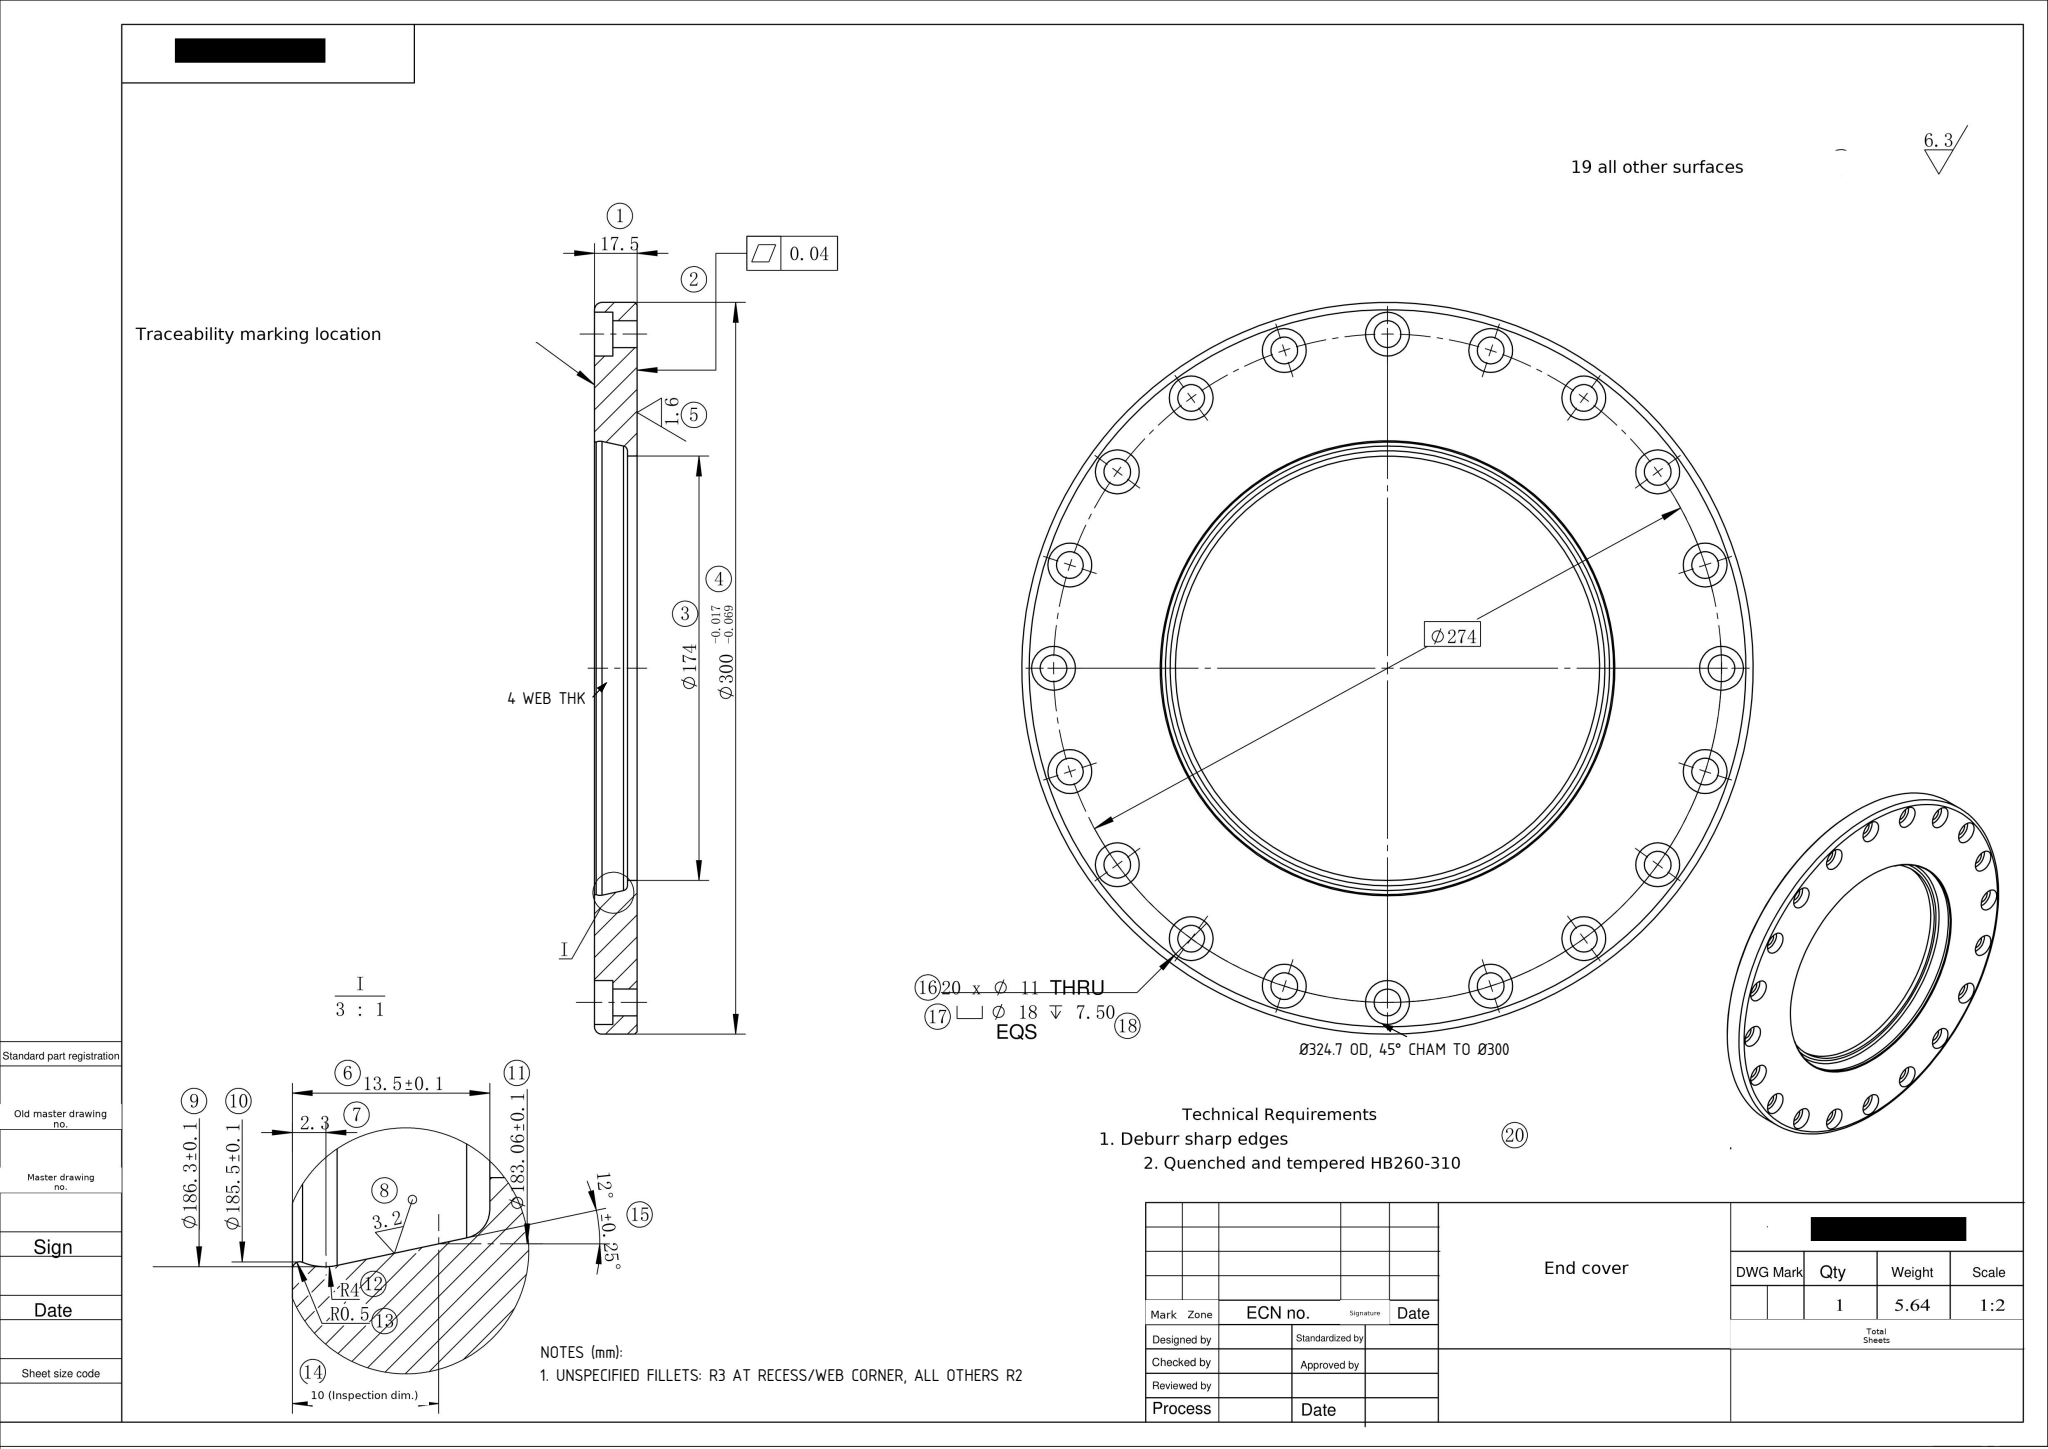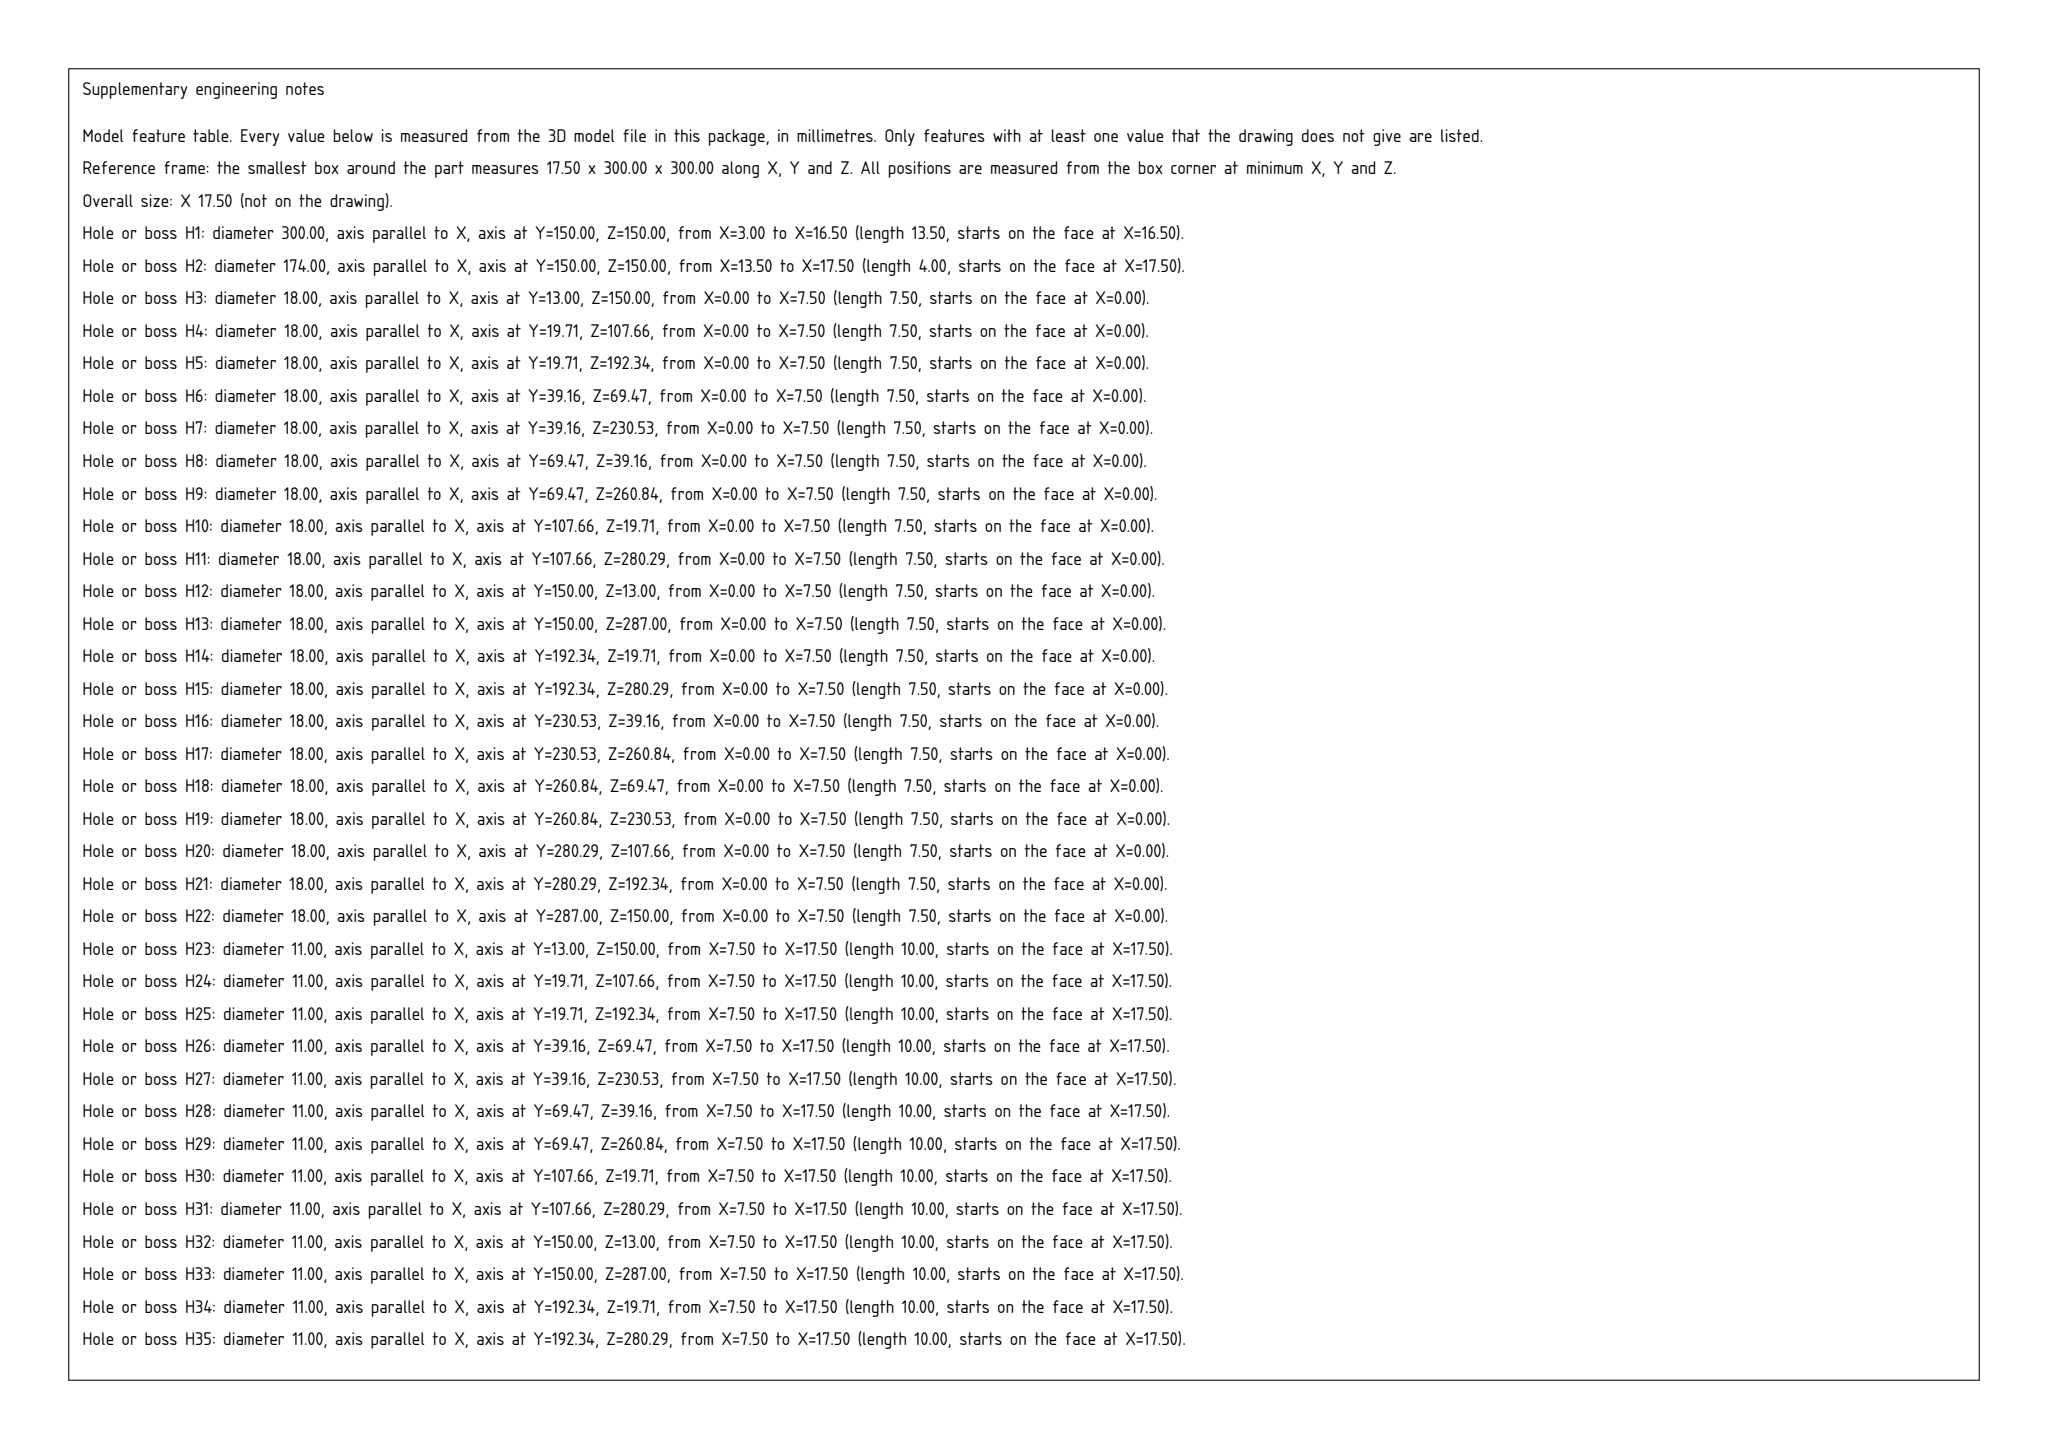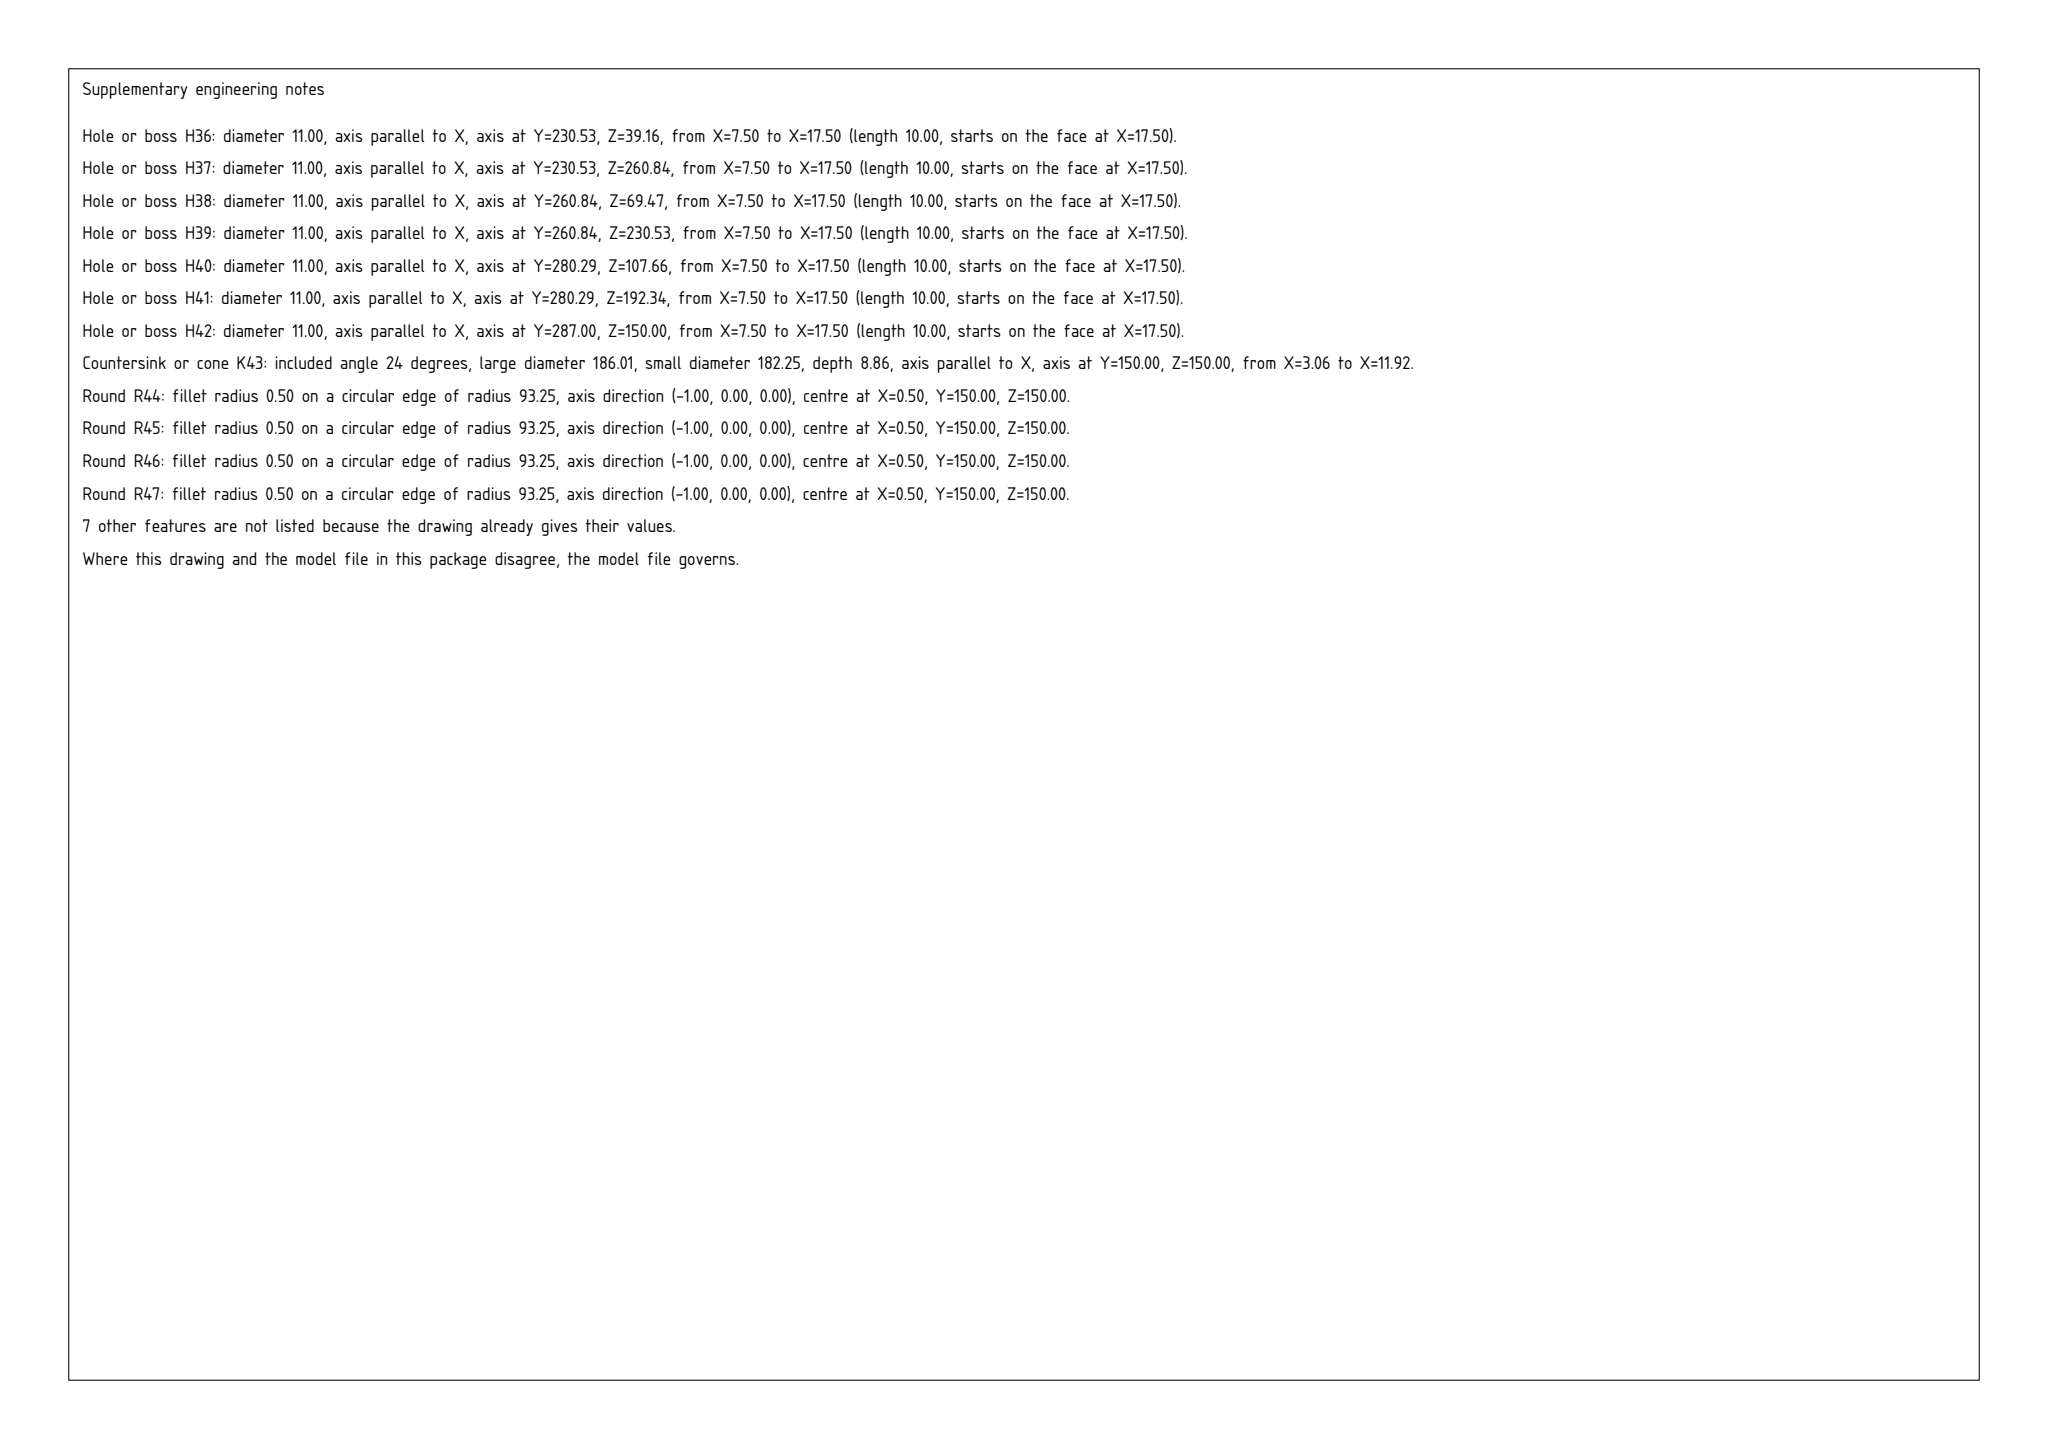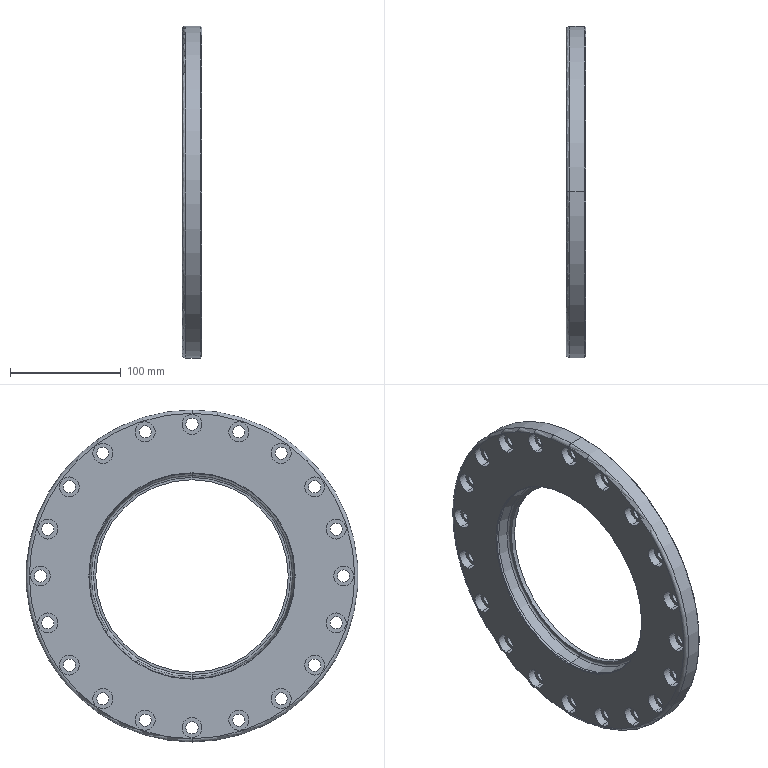Part | SolidWorks | mm | 1 solid | 121 faces | box 17.5 x 300 x 300 mm | volume 722631 mm3 | cylinder 84 | plane 23 | torus 10 | cone 4 | commonest cylinder face diameters 18 x40 11 x40 174 x2 300 x2
Drawing notes:
FLANGE OD Ø324.7; 45° CHAMFER (90° INCL) DOWN TO Ø300 | from the solid: bbox_xyz max 324.718 OD; cones [90.0, 300.0] x2 = 45° taper off Ø300 surface
WEB 4 THK BETWEEN RECESS FACE AND BACK FACE | from the solid: Planes x=14.12 (recess face) to x=18.12 (back face) = 4.0; Ø174 bore length 4.0
UNSPECIFIED FILLETS: R3 AT RECESS/WEB CORNER, ALL OTHERS R2 | from the solid: fillet_radii include [3.0,2] and [2.0,2]; R0.5 and R4 already called out in detail I
build123d program:
from build123d import *

# Parameters (mm, degrees)
HOLE_SIZE_ACCORDING_TO_HEXAGON_SOCKET_D           = 11
HOLE_SIZE_ACCORDING_TO_HEXAGON_SOCKET_CBORE_D     = 18
HOLE_SIZE_ACCORDING_TO_HEXAGON_SOCKET_CBORE_DEPTH = 7.5
CIRPATTERN1_COUNT                                 = 20
FILLET2_R                                         = 3
CHAMFER1_SIZE                                     = 1


with BuildPart() as part:
    # Sketch1 → Revolve1 (revolve)
    with BuildSketch(Plane.XY, mode=Mode.PRIVATE) as revolve1_sk:
        with BuildLine():
            Line((-1.858, -150), (15.642, -150))
            Line((15.642, -150), (15.642, -87))
            Line((15.642, -87), (11.642, -87))
            Line((11.642, -87), (11.642, -89.166))
            ThreePointArc((11.642, -89.166), (11.196, -90.425), (10.058, -91.123))
            Line((10.058, -91.123), (1.198, -93.006))
            ThreePointArc((1.198, -93.006), (-0.001041, -93.077), (-1.167, -92.788))
            ThreePointArc((-1.167, -92.788), (-1.636, -92.834), (-1.858, -93.25))
            Line((-1.858, -93.25), (-1.858, -150))
        make_face()
    revolve(revolve1_sk.sketch.rotate(Axis((0, 0, 0), (1, 0, 0)), 270), axis=Axis((0, 0, 0), (1, 0, 0)))

    # Hole Size _ according to_ Hexagon Socket (through all)
    with Locations(Plane.ZY.offset(1.858)):
        with Locations((0, 137)):
            hole_size_according_to_hexagon_socket = CounterBoreHole(HOLE_SIZE_ACCORDING_TO_HEXAGON_SOCKET_D / 2, HOLE_SIZE_ACCORDING_TO_HEXAGON_SOCKET_CBORE_D / 2, HOLE_SIZE_ACCORDING_TO_HEXAGON_SOCKET_CBORE_DEPTH)

    # CirPattern1: Hole Size _ according to_ Hexagon Socket ×20 about axis
    cirpattern1_axis = Axis((0, 0, 0), (1, 0, 0))
    for i in range(1, CIRPATTERN1_COUNT):
        add(hole_size_according_to_hexagon_socket.rotate(cirpattern1_axis, i * 360 / CIRPATTERN1_COUNT), mode=Mode.SUBTRACT)

    # Fillet2
    fillet2_edges = [part.edges().sort_by_distance(p)[0] for p in [
        (-1.858, 0, -150),
    ]]
    fillet(fillet2_edges, radius=FILLET2_R)

    # Chamfer1
    chamfer1_edges = [part.edges().sort_by_distance(p)[0] for p in [
        (15.642, 0, -150),
    ]]
    chamfer(chamfer1_edges, length=CHAMFER1_SIZE)


solid = part.part